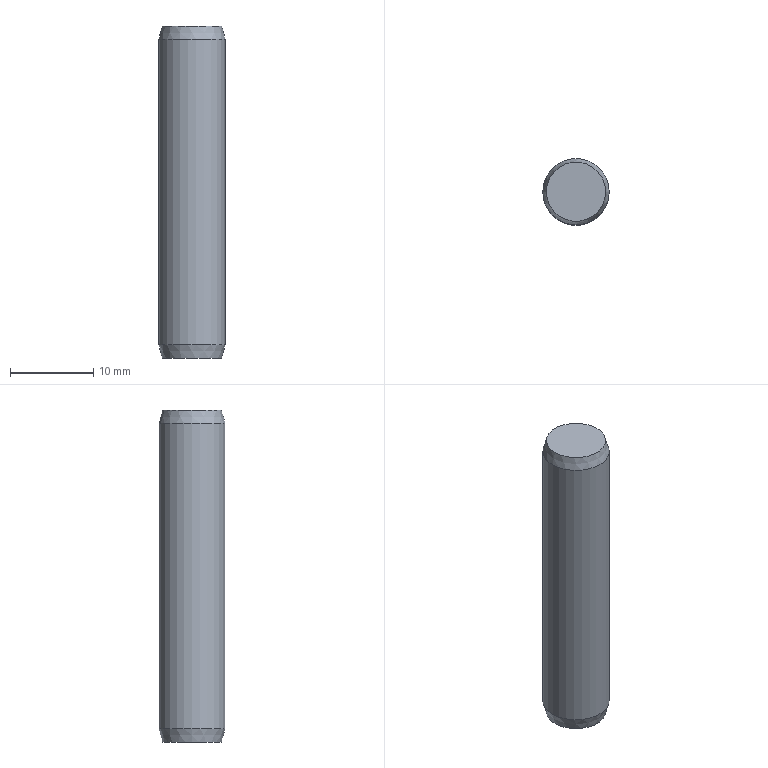Component | NX | GB-T119_1-2000_8X40 | 1 solid | 5 faces | box 8 x 8 x 40 mm | volume 1994 mm3 | plane 2 | cone 2 | cylinder 1 | commonest cylinder face diameters 8 x1
STEP:
#1=CARTESIAN_POINT('',(0.,0.,0.));
#2=DIRECTION('',(0.,0.,1.));
#3=DIRECTION('',(1.,0.,0.));
#4=AXIS2_PLACEMENT_3D('',#1,#2,#3);
#5=CARTESIAN_POINT('',(-3.571,-36.5,15.));
#6=VERTEX_POINT('',#5);
#7=CARTESIAN_POINT('',(0.,-36.5,15.));
#8=DIRECTION('',(0.,0.,-1.));
#9=DIRECTION('',(-1.,0.,0.));
#10=AXIS2_PLACEMENT_3D('',#7,#8,#9);
#11=CIRCLE('',#10,3.571);
#12=CARTESIAN_POINT('',(0.,-36.5,15.));
#13=DIRECTION('',(0.,0.,-1.));
#14=DIRECTION('',(-1.,0.,0.));
#15=AXIS2_PLACEMENT_3D('',#12,#13,#14);
#16=PLANE('',#15);
#17=CARTESIAN_POINT('',(0.,0.));
#18=DIRECTION('',(1.,0.));
#19=AXIS2_PLACEMENT_2D('',#17,#18);
#20=CIRCLE('',#19,3.571);
#21=(GEOMETRIC_REPRESENTATION_CONTEXT(2)PARAMETRIC_REPRESENTATION_CONTEXT()REPRESENTATION_CONTEXT('',''));
#22=DEFINITIONAL_REPRESENTATION('',(#20),#21);
#23=PCURVE('',#16,#22);
#24=CARTESIAN_POINT('',(0.,-36.5,15.));
#25=DIRECTION('',(0.,0.,1.));
#26=DIRECTION('',(1.,0.,0.));
#27=AXIS2_PLACEMENT_3D('',#24,#25,#26);
#28=CONICAL_SURFACE('',#27,3.571,0.2618);
#29=CARTESIAN_POINT('',(9.425,0.));
#30=DIRECTION('',(-1.,0.));
#31=VECTOR('',#30,1.);
#32=LINE('',#29,#31);
#33=(GEOMETRIC_REPRESENTATION_CONTEXT(2)PARAMETRIC_REPRESENTATION_CONTEXT()REPRESENTATION_CONTEXT('',''));
#34=DEFINITIONAL_REPRESENTATION('',(#32),#33);
#35=PCURVE('',#28,#34);
#36=SURFACE_CURVE('',#11,(#23,#35),.PCURVE_S1.);
#37=EDGE_CURVE('',#6,#6,#36,.T.);
#38=ORIENTED_EDGE('',*,*,#37,.T.);
#39=EDGE_LOOP('',(#38));
#40=FACE_BOUND('',#39,.T.);
#41=ADVANCED_FACE('',(#40),#16,.T.);
#42=CARTESIAN_POINT('',(-4.,-36.5,16.6));
#43=VERTEX_POINT('',#42);
#44=CARTESIAN_POINT('',(0.,-36.5,16.6));
#45=DIRECTION('',(0.,0.,-1.));
#46=DIRECTION('',(-1.,0.,0.));
#47=AXIS2_PLACEMENT_3D('',#44,#45,#46);
#48=CIRCLE('',#47,4.);
#49=CARTESIAN_POINT('',(9.425,1.6));
#50=DIRECTION('',(-1.,0.));
#51=VECTOR('',#50,1.);
#52=LINE('',#49,#51);
#53=(GEOMETRIC_REPRESENTATION_CONTEXT(2)PARAMETRIC_REPRESENTATION_CONTEXT()REPRESENTATION_CONTEXT('',''));
#54=DEFINITIONAL_REPRESENTATION('',(#52),#53);
#55=PCURVE('',#28,#54);
#56=CARTESIAN_POINT('',(0.,-36.5,55.));
#57=DIRECTION('',(0.,0.,-1.));
#58=DIRECTION('',(-1.,0.,0.));
#59=AXIS2_PLACEMENT_3D('',#56,#57,#58);
#60=CYLINDRICAL_SURFACE('',#59,4.);
#61=CARTESIAN_POINT('',(0.,38.4));
#62=DIRECTION('',(1.,0.));
#63=VECTOR('',#62,1.);
#64=LINE('',#61,#63);
#65=(GEOMETRIC_REPRESENTATION_CONTEXT(2)PARAMETRIC_REPRESENTATION_CONTEXT()REPRESENTATION_CONTEXT('',''));
#66=DEFINITIONAL_REPRESENTATION('',(#64),#65);
#67=PCURVE('',#60,#66);
#68=SURFACE_CURVE('',#48,(#55,#67),.PCURVE_S1.);
#69=EDGE_CURVE('',#43,#43,#68,.T.);
#70=ORIENTED_EDGE('',*,*,#69,.T.);
#71=CARTESIAN_POINT('',(-3.571,-36.5,15.));
#72=CARTESIAN_POINT('',(-4.,-36.5,16.6));
#73=B_SPLINE_CURVE_WITH_KNOTS('',1,(#71,#72),.UNSPECIFIED.,.F.,.F.,(2,2),(0.,1.656),.PIECEWISE_BEZIER_KNOTS.);
#74=CARTESIAN_POINT('',(3.142,0.));
#75=DIRECTION('',(0.,1.));
#76=VECTOR('',#75,1.);
#77=LINE('',#74,#76);
#78=(GEOMETRIC_REPRESENTATION_CONTEXT(2)PARAMETRIC_REPRESENTATION_CONTEXT()REPRESENTATION_CONTEXT('',''));
#79=DEFINITIONAL_REPRESENTATION('',(#77),#78);
#80=PCURVE('',#28,#79);
#81=CARTESIAN_POINT('',(9.425,0.));
#82=DIRECTION('',(0.,1.));
#83=VECTOR('',#82,1.);
#84=LINE('',#81,#83);
#85=(GEOMETRIC_REPRESENTATION_CONTEXT(2)PARAMETRIC_REPRESENTATION_CONTEXT()REPRESENTATION_CONTEXT('',''));
#86=DEFINITIONAL_REPRESENTATION('',(#84),#85);
#87=PCURVE('',#28,#86);
#88=SEAM_CURVE('',#73,(#80,#87),.PCURVE_S1.);
#89=EDGE_CURVE('',#6,#43,#88,.T.);
#90=ORIENTED_EDGE('',*,*,#89,.F.);
#91=ORIENTED_EDGE('',*,*,#37,.F.);
#92=ORIENTED_EDGE('',*,*,#89,.T.);
#93=EDGE_LOOP('',(#70,#90,#91,#92));
#94=FACE_BOUND('',#93,.T.);
#95=ADVANCED_FACE('',(#94),#28,.T.);
#96=CARTESIAN_POINT('',(-4.,-36.5,53.4));
#97=VERTEX_POINT('',#96);
#98=CARTESIAN_POINT('',(0.,-36.5,53.4));
#99=DIRECTION('',(0.,0.,-1.));
#100=DIRECTION('',(-1.,0.,0.));
#101=AXIS2_PLACEMENT_3D('',#98,#99,#100);
#102=CIRCLE('',#101,4.);
#103=CARTESIAN_POINT('',(0.,1.6));
#104=DIRECTION('',(1.,0.));
#105=VECTOR('',#104,1.);
#106=LINE('',#103,#105);
#107=(GEOMETRIC_REPRESENTATION_CONTEXT(2)PARAMETRIC_REPRESENTATION_CONTEXT()REPRESENTATION_CONTEXT('',''));
#108=DEFINITIONAL_REPRESENTATION('',(#106),#107);
#109=PCURVE('',#60,#108);
#110=CARTESIAN_POINT('',(0.,-36.5,53.4));
#111=DIRECTION('',(0.,0.,-1.));
#112=DIRECTION('',(-1.,0.,0.));
#113=AXIS2_PLACEMENT_3D('',#110,#111,#112);
#114=CONICAL_SURFACE('',#113,4.,0.2618);
#115=CARTESIAN_POINT('',(0.,0.));
#116=DIRECTION('',(1.,0.));
#117=VECTOR('',#116,1.);
#118=LINE('',#115,#117);
#119=(GEOMETRIC_REPRESENTATION_CONTEXT(2)PARAMETRIC_REPRESENTATION_CONTEXT()REPRESENTATION_CONTEXT('',''));
#120=DEFINITIONAL_REPRESENTATION('',(#118),#119);
#121=PCURVE('',#114,#120);
#122=SURFACE_CURVE('',#102,(#109,#121),.PCURVE_S1.);
#123=EDGE_CURVE('',#97,#97,#122,.T.);
#124=ORIENTED_EDGE('',*,*,#123,.T.);
#125=CARTESIAN_POINT('',(-4.,-36.5,53.4));
#126=CARTESIAN_POINT('',(-4.,-36.5,16.6));
#127=B_SPLINE_CURVE_WITH_KNOTS('',1,(#125,#126),.UNSPECIFIED.,.F.,.F.,(2,2),(1.6,38.4),.PIECEWISE_BEZIER_KNOTS.);
#128=CARTESIAN_POINT('',(6.283,0.));
#129=DIRECTION('',(0.,1.));
#130=VECTOR('',#129,1.);
#131=LINE('',#128,#130);
#132=(GEOMETRIC_REPRESENTATION_CONTEXT(2)PARAMETRIC_REPRESENTATION_CONTEXT()REPRESENTATION_CONTEXT('',''));
#133=DEFINITIONAL_REPRESENTATION('',(#131),#132);
#134=PCURVE('',#60,#133);
#135=CARTESIAN_POINT('',(0.,0.));
#136=DIRECTION('',(0.,1.));
#137=VECTOR('',#136,1.);
#138=LINE('',#135,#137);
#139=(GEOMETRIC_REPRESENTATION_CONTEXT(2)PARAMETRIC_REPRESENTATION_CONTEXT()REPRESENTATION_CONTEXT('',''));
#140=DEFINITIONAL_REPRESENTATION('',(#138),#139);
#141=PCURVE('',#60,#140);
#142=SEAM_CURVE('',#127,(#134,#141),.PCURVE_S1.);
#143=EDGE_CURVE('',#97,#43,#142,.T.);
#144=ORIENTED_EDGE('',*,*,#143,.T.);
#145=ORIENTED_EDGE('',*,*,#69,.F.);
#146=ORIENTED_EDGE('',*,*,#143,.F.);
#147=EDGE_LOOP('',(#124,#144,#145,#146));
#148=FACE_BOUND('',#147,.T.);
#149=ADVANCED_FACE('',(#148),#60,.T.);
#150=CARTESIAN_POINT('',(-3.571,-36.5,55.));
#151=VERTEX_POINT('',#150);
#152=CARTESIAN_POINT('',(0.,-36.5,55.));
#153=DIRECTION('',(0.,0.,-1.));
#154=DIRECTION('',(-1.,0.,0.));
#155=AXIS2_PLACEMENT_3D('',#152,#153,#154);
#156=CIRCLE('',#155,3.571);
#157=CARTESIAN_POINT('',(0.,-1.6));
#158=DIRECTION('',(1.,0.));
#159=VECTOR('',#158,1.);
#160=LINE('',#157,#159);
#161=(GEOMETRIC_REPRESENTATION_CONTEXT(2)PARAMETRIC_REPRESENTATION_CONTEXT()REPRESENTATION_CONTEXT('',''));
#162=DEFINITIONAL_REPRESENTATION('',(#160),#161);
#163=PCURVE('',#114,#162);
#164=CARTESIAN_POINT('',(3.571,-36.5,55.));
#165=DIRECTION('',(0.,0.,1.));
#166=DIRECTION('',(1.,0.,0.));
#167=AXIS2_PLACEMENT_3D('',#164,#165,#166);
#168=PLANE('',#167);
#169=CARTESIAN_POINT('',(-7.143,0.));
#170=CARTESIAN_POINT('',(-7.143,6.186));
#171=CARTESIAN_POINT('',(-1.786,3.093));
#172=CARTESIAN_POINT('',(3.571,0.));
#173=CARTESIAN_POINT('',(-1.786,-3.093));
#174=CARTESIAN_POINT('',(-7.143,-6.186));
#175=CARTESIAN_POINT('',(-7.143,0.));
#176=(BOUNDED_CURVE()B_SPLINE_CURVE(2,(#169,#170,#171,#172,#173,#174,#175),.UNSPECIFIED.,.T.,.F.)B_SPLINE_CURVE_WITH_KNOTS((1,2,2,2,2,1),(-2.094,0.,2.094,4.189,6.283,8.378),.UNSPECIFIED.)CURVE()GEOMETRIC_REPRESENTATION_ITEM()RATIONAL_B_SPLINE_CURVE((1.,0.5,1.,0.5,1.,0.5,1.))REPRESENTATION_ITEM(''));
#177=(GEOMETRIC_REPRESENTATION_CONTEXT(2)PARAMETRIC_REPRESENTATION_CONTEXT()REPRESENTATION_CONTEXT('',''));
#178=DEFINITIONAL_REPRESENTATION('',(#176),#177);
#179=PCURVE('',#168,#178);
#180=SURFACE_CURVE('',#156,(#163,#179),.PCURVE_S1.);
#181=EDGE_CURVE('',#151,#151,#180,.T.);
#182=ORIENTED_EDGE('',*,*,#181,.T.);
#183=CARTESIAN_POINT('',(-3.571,-36.5,55.));
#184=CARTESIAN_POINT('',(-4.,-36.5,53.4));
#185=B_SPLINE_CURVE_WITH_KNOTS('',1,(#183,#184),.UNSPECIFIED.,.F.,.F.,(2,2),(-1.656,0.),.PIECEWISE_BEZIER_KNOTS.);
#186=CARTESIAN_POINT('',(6.283,0.));
#187=DIRECTION('',(0.,1.));
#188=VECTOR('',#187,1.);
#189=LINE('',#186,#188);
#190=(GEOMETRIC_REPRESENTATION_CONTEXT(2)PARAMETRIC_REPRESENTATION_CONTEXT()REPRESENTATION_CONTEXT('',''));
#191=DEFINITIONAL_REPRESENTATION('',(#189),#190);
#192=PCURVE('',#114,#191);
#193=CARTESIAN_POINT('',(0.,0.));
#194=DIRECTION('',(0.,1.));
#195=VECTOR('',#194,1.);
#196=LINE('',#193,#195);
#197=(GEOMETRIC_REPRESENTATION_CONTEXT(2)PARAMETRIC_REPRESENTATION_CONTEXT()REPRESENTATION_CONTEXT('',''));
#198=DEFINITIONAL_REPRESENTATION('',(#196),#197);
#199=PCURVE('',#114,#198);
#200=SEAM_CURVE('',#185,(#192,#199),.PCURVE_S1.);
#201=EDGE_CURVE('',#151,#97,#200,.T.);
#202=ORIENTED_EDGE('',*,*,#201,.T.);
#203=ORIENTED_EDGE('',*,*,#123,.F.);
#204=ORIENTED_EDGE('',*,*,#201,.F.);
#205=EDGE_LOOP('',(#182,#202,#203,#204));
#206=FACE_BOUND('',#205,.T.);
#207=ADVANCED_FACE('',(#206),#114,.T.);
#208=ORIENTED_EDGE('',*,*,#181,.F.);
#209=EDGE_LOOP('',(#208));
#210=FACE_BOUND('',#209,.T.);
#211=ADVANCED_FACE('',(#210),#168,.T.);
#212=CLOSED_SHELL('',(#41,#95,#149,#207,#211));
#213=MANIFOLD_SOLID_BREP('',#212);
#214=(LENGTH_UNIT()NAMED_UNIT(*)SI_UNIT(.MILLI.,.METRE.));
#215=UNCERTAINTY_MEASURE_WITH_UNIT(LENGTH_MEASURE(0.00001),#214,'','');
#216=(NAMED_UNIT(*)PLANE_ANGLE_UNIT()SI_UNIT($,.RADIAN.));
#217=(NAMED_UNIT(*)SI_UNIT($,.STERADIAN.)SOLID_ANGLE_UNIT());
#218=(GEOMETRIC_REPRESENTATION_CONTEXT(3)GLOBAL_UNCERTAINTY_ASSIGNED_CONTEXT((#215))GLOBAL_UNIT_ASSIGNED_CONTEXT((#214,#216,#217))REPRESENTATION_CONTEXT('',''));
#219=ADVANCED_BREP_SHAPE_REPRESENTATION('',(#4,#213),#218);